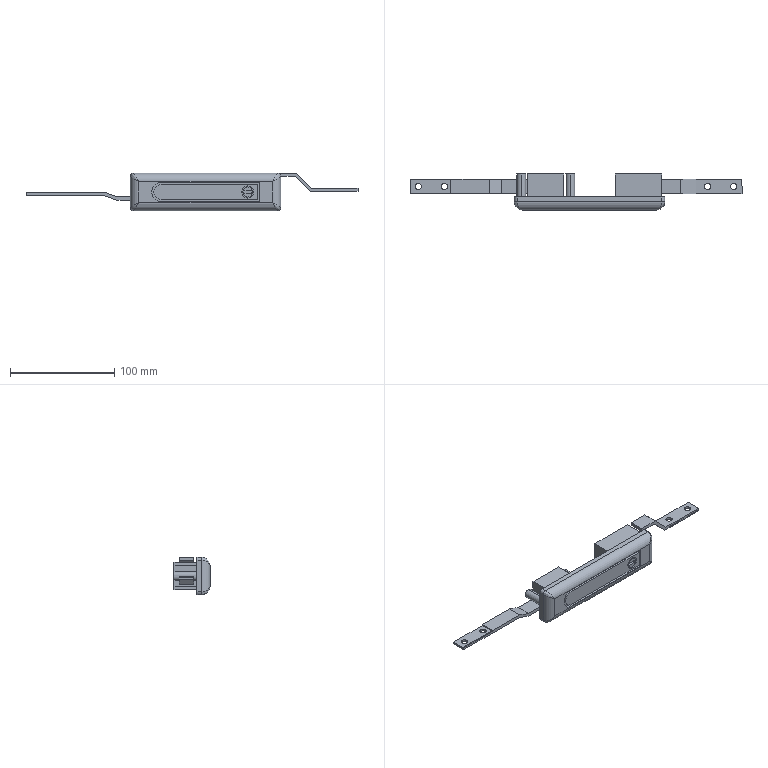Component | SolidWorks | FrontDoorAssembly-1_Lock(MS828)-1 | 2 solids | 91 faces | volume 109162 mm3 | plane 59 | cylinder 28 | spline 4 | commonest cylinder face diameters 6 x12 8.5 x4 16 x4 4 x2 11.658 x2 9.658 x2 19.043 x1 15.043 x1